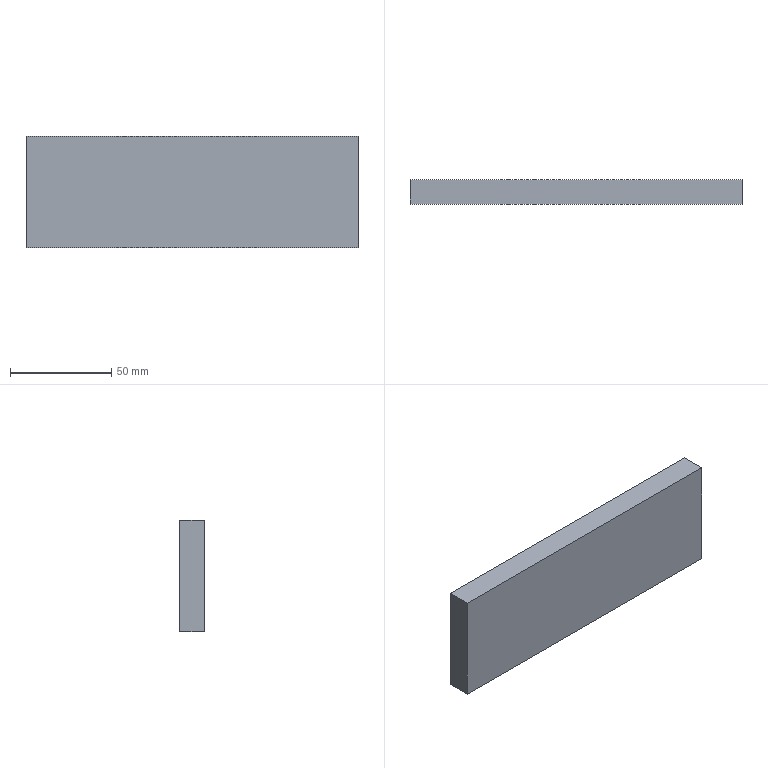Component | NX | CH3404_5-4 | 1 solid | 6 faces | box 164 x 12 x 55 mm | volume 108240 mm3 | plane 6
STEP:
#1=CARTESIAN_POINT('',(0.,0.,0.));
#2=DIRECTION('',(0.,0.,1.));
#3=DIRECTION('',(1.,0.,0.));
#4=AXIS2_PLACEMENT_3D('',#1,#2,#3);
#5=CARTESIAN_POINT('',(115.,-6.,-55.));
#6=VERTEX_POINT('',#5);
#7=CARTESIAN_POINT('',(115.,-6.,-0.));
#8=VERTEX_POINT('',#7);
#9=CARTESIAN_POINT('',(115.,-6.,-55.));
#10=DIRECTION('',(0.,0.,1.));
#11=VECTOR('',#10,1.);
#12=LINE('',#9,#11);
#13=CARTESIAN_POINT('',(115.,6.,-55.));
#14=DIRECTION('',(1.,0.,0.));
#15=DIRECTION('',(0.,0.,-1.));
#16=AXIS2_PLACEMENT_3D('',#13,#14,#15);
#17=PLANE('',#16);
#18=CARTESIAN_POINT('',(0.,-12.));
#19=DIRECTION('',(-1.,0.));
#20=VECTOR('',#19,1.);
#21=LINE('',#18,#20);
#22=(GEOMETRIC_REPRESENTATION_CONTEXT(2)PARAMETRIC_REPRESENTATION_CONTEXT()REPRESENTATION_CONTEXT('',''));
#23=DEFINITIONAL_REPRESENTATION('',(#21),#22);
#24=PCURVE('',#17,#23);
#25=CARTESIAN_POINT('',(197.,-6.,-27.5));
#26=DIRECTION('',(0.,1.,0.));
#27=DIRECTION('',(0.,0.,1.));
#28=AXIS2_PLACEMENT_3D('',#25,#26,#27);
#29=PLANE('',#28);
#30=CARTESIAN_POINT('',(-27.5,-82.));
#31=DIRECTION('',(1.,0.));
#32=VECTOR('',#31,1.);
#33=LINE('',#30,#32);
#34=(GEOMETRIC_REPRESENTATION_CONTEXT(2)PARAMETRIC_REPRESENTATION_CONTEXT()REPRESENTATION_CONTEXT('',''));
#35=DEFINITIONAL_REPRESENTATION('',(#33),#34);
#36=PCURVE('',#29,#35);
#37=SURFACE_CURVE('',#12,(#24,#36),.PCURVE_S1.);
#38=EDGE_CURVE('',#6,#8,#37,.T.);
#39=ORIENTED_EDGE('',*,*,#38,.T.);
#40=CARTESIAN_POINT('',(115.,6.,-0.));
#41=VERTEX_POINT('',#40);
#42=CARTESIAN_POINT('',(115.,6.,-0.));
#43=DIRECTION('',(0.,-1.,0.));
#44=VECTOR('',#43,1.);
#45=LINE('',#42,#44);
#46=CARTESIAN_POINT('',(-55.,0.));
#47=DIRECTION('',(0.,-1.));
#48=VECTOR('',#47,1.);
#49=LINE('',#46,#48);
#50=(GEOMETRIC_REPRESENTATION_CONTEXT(2)PARAMETRIC_REPRESENTATION_CONTEXT()REPRESENTATION_CONTEXT('',''));
#51=DEFINITIONAL_REPRESENTATION('',(#49),#50);
#52=PCURVE('',#17,#51);
#53=CARTESIAN_POINT('',(115.,6.,-0.));
#54=DIRECTION('',(0.,0.,-1.));
#55=DIRECTION('',(-1.,0.,-0.));
#56=AXIS2_PLACEMENT_3D('',#53,#54,#55);
#57=PLANE('',#56);
#58=CARTESIAN_POINT('',(0.,0.));
#59=DIRECTION('',(0.,-1.));
#60=VECTOR('',#59,1.);
#61=LINE('',#58,#60);
#62=(GEOMETRIC_REPRESENTATION_CONTEXT(2)PARAMETRIC_REPRESENTATION_CONTEXT()REPRESENTATION_CONTEXT('',''));
#63=DEFINITIONAL_REPRESENTATION('',(#61),#62);
#64=PCURVE('',#57,#63);
#65=SURFACE_CURVE('',#45,(#52,#64),.PCURVE_S1.);
#66=EDGE_CURVE('',#41,#8,#65,.T.);
#67=ORIENTED_EDGE('',*,*,#66,.F.);
#68=CARTESIAN_POINT('',(115.,6.,-55.));
#69=VERTEX_POINT('',#68);
#70=CARTESIAN_POINT('',(115.,6.,-55.));
#71=DIRECTION('',(0.,0.,1.));
#72=VECTOR('',#71,1.);
#73=LINE('',#70,#72);
#74=CARTESIAN_POINT('',(0.,0.));
#75=DIRECTION('',(-1.,0.));
#76=VECTOR('',#75,1.);
#77=LINE('',#74,#76);
#78=(GEOMETRIC_REPRESENTATION_CONTEXT(2)PARAMETRIC_REPRESENTATION_CONTEXT()REPRESENTATION_CONTEXT('',''));
#79=DEFINITIONAL_REPRESENTATION('',(#77),#78);
#80=PCURVE('',#17,#79);
#81=CARTESIAN_POINT('',(197.,6.,-27.5));
#82=DIRECTION('',(0.,1.,0.));
#83=DIRECTION('',(0.,0.,1.));
#84=AXIS2_PLACEMENT_3D('',#81,#82,#83);
#85=PLANE('',#84);
#86=CARTESIAN_POINT('',(-27.5,-82.));
#87=DIRECTION('',(1.,0.));
#88=VECTOR('',#87,1.);
#89=LINE('',#86,#88);
#90=(GEOMETRIC_REPRESENTATION_CONTEXT(2)PARAMETRIC_REPRESENTATION_CONTEXT()REPRESENTATION_CONTEXT('',''));
#91=DEFINITIONAL_REPRESENTATION('',(#89),#90);
#92=PCURVE('',#85,#91);
#93=SURFACE_CURVE('',#73,(#80,#92),.PCURVE_S1.);
#94=EDGE_CURVE('',#69,#41,#93,.T.);
#95=ORIENTED_EDGE('',*,*,#94,.F.);
#96=CARTESIAN_POINT('',(115.,6.,-55.));
#97=DIRECTION('',(0.,-1.,0.));
#98=VECTOR('',#97,1.);
#99=LINE('',#96,#98);
#100=CARTESIAN_POINT('',(0.,0.));
#101=DIRECTION('',(0.,-1.));
#102=VECTOR('',#101,1.);
#103=LINE('',#100,#102);
#104=(GEOMETRIC_REPRESENTATION_CONTEXT(2)PARAMETRIC_REPRESENTATION_CONTEXT()REPRESENTATION_CONTEXT('',''));
#105=DEFINITIONAL_REPRESENTATION('',(#103),#104);
#106=PCURVE('',#17,#105);
#107=CARTESIAN_POINT('',(279.,6.,-55.));
#108=DIRECTION('',(0.,0.,1.));
#109=DIRECTION('',(1.,0.,-0.));
#110=AXIS2_PLACEMENT_3D('',#107,#108,#109);
#111=PLANE('',#110);
#112=CARTESIAN_POINT('',(-164.,0.));
#113=DIRECTION('',(0.,-1.));
#114=VECTOR('',#113,1.);
#115=LINE('',#112,#114);
#116=(GEOMETRIC_REPRESENTATION_CONTEXT(2)PARAMETRIC_REPRESENTATION_CONTEXT()REPRESENTATION_CONTEXT('',''));
#117=DEFINITIONAL_REPRESENTATION('',(#115),#116);
#118=PCURVE('',#111,#117);
#119=SURFACE_CURVE('',#99,(#106,#118),.PCURVE_S1.);
#120=EDGE_CURVE('',#69,#6,#119,.T.);
#121=ORIENTED_EDGE('',*,*,#120,.T.);
#122=EDGE_LOOP('',(#39,#67,#95,#121));
#123=FACE_BOUND('',#122,.T.);
#124=ADVANCED_FACE('',(#123),#17,.F.);
#125=CARTESIAN_POINT('',(279.,-6.,-0.));
#126=VERTEX_POINT('',#125);
#127=CARTESIAN_POINT('',(115.,-6.,-0.));
#128=DIRECTION('',(1.,0.,0.));
#129=VECTOR('',#128,1.);
#130=LINE('',#127,#129);
#131=CARTESIAN_POINT('',(0.,-12.));
#132=DIRECTION('',(-1.,0.));
#133=VECTOR('',#132,1.);
#134=LINE('',#131,#133);
#135=(GEOMETRIC_REPRESENTATION_CONTEXT(2)PARAMETRIC_REPRESENTATION_CONTEXT()REPRESENTATION_CONTEXT('',''));
#136=DEFINITIONAL_REPRESENTATION('',(#134),#135);
#137=PCURVE('',#57,#136);
#138=CARTESIAN_POINT('',(27.5,-82.));
#139=DIRECTION('',(0.,1.));
#140=VECTOR('',#139,1.);
#141=LINE('',#138,#140);
#142=(GEOMETRIC_REPRESENTATION_CONTEXT(2)PARAMETRIC_REPRESENTATION_CONTEXT()REPRESENTATION_CONTEXT('',''));
#143=DEFINITIONAL_REPRESENTATION('',(#141),#142);
#144=PCURVE('',#29,#143);
#145=SURFACE_CURVE('',#130,(#137,#144),.PCURVE_S1.);
#146=EDGE_CURVE('',#8,#126,#145,.T.);
#147=ORIENTED_EDGE('',*,*,#146,.T.);
#148=CARTESIAN_POINT('',(279.,6.,-0.));
#149=VERTEX_POINT('',#148);
#150=CARTESIAN_POINT('',(279.,6.,-0.));
#151=DIRECTION('',(0.,-1.,0.));
#152=VECTOR('',#151,1.);
#153=LINE('',#150,#152);
#154=CARTESIAN_POINT('',(-164.,0.));
#155=DIRECTION('',(0.,-1.));
#156=VECTOR('',#155,1.);
#157=LINE('',#154,#156);
#158=(GEOMETRIC_REPRESENTATION_CONTEXT(2)PARAMETRIC_REPRESENTATION_CONTEXT()REPRESENTATION_CONTEXT('',''));
#159=DEFINITIONAL_REPRESENTATION('',(#157),#158);
#160=PCURVE('',#57,#159);
#161=CARTESIAN_POINT('',(279.,6.,-0.));
#162=DIRECTION('',(-1.,0.,0.));
#163=DIRECTION('',(0.,0.,1.));
#164=AXIS2_PLACEMENT_3D('',#161,#162,#163);
#165=PLANE('',#164);
#166=CARTESIAN_POINT('',(0.,0.));
#167=DIRECTION('',(0.,-1.));
#168=VECTOR('',#167,1.);
#169=LINE('',#166,#168);
#170=(GEOMETRIC_REPRESENTATION_CONTEXT(2)PARAMETRIC_REPRESENTATION_CONTEXT()REPRESENTATION_CONTEXT('',''));
#171=DEFINITIONAL_REPRESENTATION('',(#169),#170);
#172=PCURVE('',#165,#171);
#173=SURFACE_CURVE('',#153,(#160,#172),.PCURVE_S1.);
#174=EDGE_CURVE('',#149,#126,#173,.T.);
#175=ORIENTED_EDGE('',*,*,#174,.F.);
#176=CARTESIAN_POINT('',(115.,6.,-0.));
#177=DIRECTION('',(1.,0.,0.));
#178=VECTOR('',#177,1.);
#179=LINE('',#176,#178);
#180=CARTESIAN_POINT('',(0.,0.));
#181=DIRECTION('',(-1.,0.));
#182=VECTOR('',#181,1.);
#183=LINE('',#180,#182);
#184=(GEOMETRIC_REPRESENTATION_CONTEXT(2)PARAMETRIC_REPRESENTATION_CONTEXT()REPRESENTATION_CONTEXT('',''));
#185=DEFINITIONAL_REPRESENTATION('',(#183),#184);
#186=PCURVE('',#57,#185);
#187=CARTESIAN_POINT('',(27.5,-82.));
#188=DIRECTION('',(0.,1.));
#189=VECTOR('',#188,1.);
#190=LINE('',#187,#189);
#191=(GEOMETRIC_REPRESENTATION_CONTEXT(2)PARAMETRIC_REPRESENTATION_CONTEXT()REPRESENTATION_CONTEXT('',''));
#192=DEFINITIONAL_REPRESENTATION('',(#190),#191);
#193=PCURVE('',#85,#192);
#194=SURFACE_CURVE('',#179,(#186,#193),.PCURVE_S1.);
#195=EDGE_CURVE('',#41,#149,#194,.T.);
#196=ORIENTED_EDGE('',*,*,#195,.F.);
#197=ORIENTED_EDGE('',*,*,#66,.T.);
#198=EDGE_LOOP('',(#147,#175,#196,#197));
#199=FACE_BOUND('',#198,.T.);
#200=ADVANCED_FACE('',(#199),#57,.F.);
#201=CARTESIAN_POINT('',(279.,-6.,-55.));
#202=VERTEX_POINT('',#201);
#203=CARTESIAN_POINT('',(279.,-6.,-0.));
#204=DIRECTION('',(-0.,0.,-1.));
#205=VECTOR('',#204,1.);
#206=LINE('',#203,#205);
#207=CARTESIAN_POINT('',(0.,-12.));
#208=DIRECTION('',(-1.,0.));
#209=VECTOR('',#208,1.);
#210=LINE('',#207,#209);
#211=(GEOMETRIC_REPRESENTATION_CONTEXT(2)PARAMETRIC_REPRESENTATION_CONTEXT()REPRESENTATION_CONTEXT('',''));
#212=DEFINITIONAL_REPRESENTATION('',(#210),#211);
#213=PCURVE('',#165,#212);
#214=CARTESIAN_POINT('',(27.5,82.));
#215=DIRECTION('',(-1.,-0.));
#216=VECTOR('',#215,1.);
#217=LINE('',#214,#216);
#218=(GEOMETRIC_REPRESENTATION_CONTEXT(2)PARAMETRIC_REPRESENTATION_CONTEXT()REPRESENTATION_CONTEXT('',''));
#219=DEFINITIONAL_REPRESENTATION('',(#217),#218);
#220=PCURVE('',#29,#219);
#221=SURFACE_CURVE('',#206,(#213,#220),.PCURVE_S1.);
#222=EDGE_CURVE('',#126,#202,#221,.T.);
#223=ORIENTED_EDGE('',*,*,#222,.T.);
#224=CARTESIAN_POINT('',(279.,6.,-55.));
#225=VERTEX_POINT('',#224);
#226=CARTESIAN_POINT('',(279.,6.,-55.));
#227=DIRECTION('',(0.,-1.,0.));
#228=VECTOR('',#227,1.);
#229=LINE('',#226,#228);
#230=CARTESIAN_POINT('',(-55.,0.));
#231=DIRECTION('',(0.,-1.));
#232=VECTOR('',#231,1.);
#233=LINE('',#230,#232);
#234=(GEOMETRIC_REPRESENTATION_CONTEXT(2)PARAMETRIC_REPRESENTATION_CONTEXT()REPRESENTATION_CONTEXT('',''));
#235=DEFINITIONAL_REPRESENTATION('',(#233),#234);
#236=PCURVE('',#165,#235);
#237=CARTESIAN_POINT('',(0.,0.));
#238=DIRECTION('',(0.,-1.));
#239=VECTOR('',#238,1.);
#240=LINE('',#237,#239);
#241=(GEOMETRIC_REPRESENTATION_CONTEXT(2)PARAMETRIC_REPRESENTATION_CONTEXT()REPRESENTATION_CONTEXT('',''));
#242=DEFINITIONAL_REPRESENTATION('',(#240),#241);
#243=PCURVE('',#111,#242);
#244=SURFACE_CURVE('',#229,(#236,#243),.PCURVE_S1.);
#245=EDGE_CURVE('',#225,#202,#244,.T.);
#246=ORIENTED_EDGE('',*,*,#245,.F.);
#247=CARTESIAN_POINT('',(279.,6.,-0.));
#248=DIRECTION('',(-0.,0.,-1.));
#249=VECTOR('',#248,1.);
#250=LINE('',#247,#249);
#251=CARTESIAN_POINT('',(0.,0.));
#252=DIRECTION('',(-1.,0.));
#253=VECTOR('',#252,1.);
#254=LINE('',#251,#253);
#255=(GEOMETRIC_REPRESENTATION_CONTEXT(2)PARAMETRIC_REPRESENTATION_CONTEXT()REPRESENTATION_CONTEXT('',''));
#256=DEFINITIONAL_REPRESENTATION('',(#254),#255);
#257=PCURVE('',#165,#256);
#258=CARTESIAN_POINT('',(27.5,82.));
#259=DIRECTION('',(-1.,-0.));
#260=VECTOR('',#259,1.);
#261=LINE('',#258,#260);
#262=(GEOMETRIC_REPRESENTATION_CONTEXT(2)PARAMETRIC_REPRESENTATION_CONTEXT()REPRESENTATION_CONTEXT('',''));
#263=DEFINITIONAL_REPRESENTATION('',(#261),#262);
#264=PCURVE('',#85,#263);
#265=SURFACE_CURVE('',#250,(#257,#264),.PCURVE_S1.);
#266=EDGE_CURVE('',#149,#225,#265,.T.);
#267=ORIENTED_EDGE('',*,*,#266,.F.);
#268=ORIENTED_EDGE('',*,*,#174,.T.);
#269=EDGE_LOOP('',(#223,#246,#267,#268));
#270=FACE_BOUND('',#269,.T.);
#271=ADVANCED_FACE('',(#270),#165,.F.);
#272=CARTESIAN_POINT('',(279.,-6.,-55.));
#273=DIRECTION('',(-1.,0.,0.));
#274=VECTOR('',#273,1.);
#275=LINE('',#272,#274);
#276=CARTESIAN_POINT('',(0.,-12.));
#277=DIRECTION('',(-1.,0.));
#278=VECTOR('',#277,1.);
#279=LINE('',#276,#278);
#280=(GEOMETRIC_REPRESENTATION_CONTEXT(2)PARAMETRIC_REPRESENTATION_CONTEXT()REPRESENTATION_CONTEXT('',''));
#281=DEFINITIONAL_REPRESENTATION('',(#279),#280);
#282=PCURVE('',#111,#281);
#283=CARTESIAN_POINT('',(-27.5,82.));
#284=DIRECTION('',(0.,-1.));
#285=VECTOR('',#284,1.);
#286=LINE('',#283,#285);
#287=(GEOMETRIC_REPRESENTATION_CONTEXT(2)PARAMETRIC_REPRESENTATION_CONTEXT()REPRESENTATION_CONTEXT('',''));
#288=DEFINITIONAL_REPRESENTATION('',(#286),#287);
#289=PCURVE('',#29,#288);
#290=SURFACE_CURVE('',#275,(#282,#289),.PCURVE_S1.);
#291=EDGE_CURVE('',#202,#6,#290,.T.);
#292=ORIENTED_EDGE('',*,*,#291,.T.);
#293=ORIENTED_EDGE('',*,*,#120,.F.);
#294=CARTESIAN_POINT('',(279.,6.,-55.));
#295=DIRECTION('',(-1.,0.,0.));
#296=VECTOR('',#295,1.);
#297=LINE('',#294,#296);
#298=CARTESIAN_POINT('',(0.,0.));
#299=DIRECTION('',(-1.,0.));
#300=VECTOR('',#299,1.);
#301=LINE('',#298,#300);
#302=(GEOMETRIC_REPRESENTATION_CONTEXT(2)PARAMETRIC_REPRESENTATION_CONTEXT()REPRESENTATION_CONTEXT('',''));
#303=DEFINITIONAL_REPRESENTATION('',(#301),#302);
#304=PCURVE('',#111,#303);
#305=CARTESIAN_POINT('',(-27.5,82.));
#306=DIRECTION('',(0.,-1.));
#307=VECTOR('',#306,1.);
#308=LINE('',#305,#307);
#309=(GEOMETRIC_REPRESENTATION_CONTEXT(2)PARAMETRIC_REPRESENTATION_CONTEXT()REPRESENTATION_CONTEXT('',''));
#310=DEFINITIONAL_REPRESENTATION('',(#308),#309);
#311=PCURVE('',#85,#310);
#312=SURFACE_CURVE('',#297,(#304,#311),.PCURVE_S1.);
#313=EDGE_CURVE('',#225,#69,#312,.T.);
#314=ORIENTED_EDGE('',*,*,#313,.F.);
#315=ORIENTED_EDGE('',*,*,#245,.T.);
#316=EDGE_LOOP('',(#292,#293,#314,#315));
#317=FACE_BOUND('',#316,.T.);
#318=ADVANCED_FACE('',(#317),#111,.F.);
#319=ORIENTED_EDGE('',*,*,#94,.T.);
#320=ORIENTED_EDGE('',*,*,#195,.T.);
#321=ORIENTED_EDGE('',*,*,#266,.T.);
#322=ORIENTED_EDGE('',*,*,#313,.T.);
#323=EDGE_LOOP('',(#319,#320,#321,#322));
#324=FACE_BOUND('',#323,.T.);
#325=ADVANCED_FACE('',(#324),#85,.T.);
#326=ORIENTED_EDGE('',*,*,#38,.F.);
#327=ORIENTED_EDGE('',*,*,#291,.F.);
#328=ORIENTED_EDGE('',*,*,#222,.F.);
#329=ORIENTED_EDGE('',*,*,#146,.F.);
#330=EDGE_LOOP('',(#326,#327,#328,#329));
#331=FACE_BOUND('',#330,.T.);
#332=ADVANCED_FACE('',(#331),#29,.F.);
#333=CLOSED_SHELL('',(#124,#200,#271,#318,#325,#332));
#334=MANIFOLD_SOLID_BREP('',#333);
#335=(LENGTH_UNIT()NAMED_UNIT(*)SI_UNIT(.MILLI.,.METRE.));
#336=UNCERTAINTY_MEASURE_WITH_UNIT(LENGTH_MEASURE(0.0000001),#335,'','');
#337=(NAMED_UNIT(*)PLANE_ANGLE_UNIT()SI_UNIT($,.RADIAN.));
#338=(NAMED_UNIT(*)SI_UNIT($,.STERADIAN.)SOLID_ANGLE_UNIT());
#339=(GEOMETRIC_REPRESENTATION_CONTEXT(3)GLOBAL_UNCERTAINTY_ASSIGNED_CONTEXT((#336))GLOBAL_UNIT_ASSIGNED_CONTEXT((#335,#337,#338))REPRESENTATION_CONTEXT('',''));
#340=ADVANCED_BREP_SHAPE_REPRESENTATION('',(#4,#334),#339);